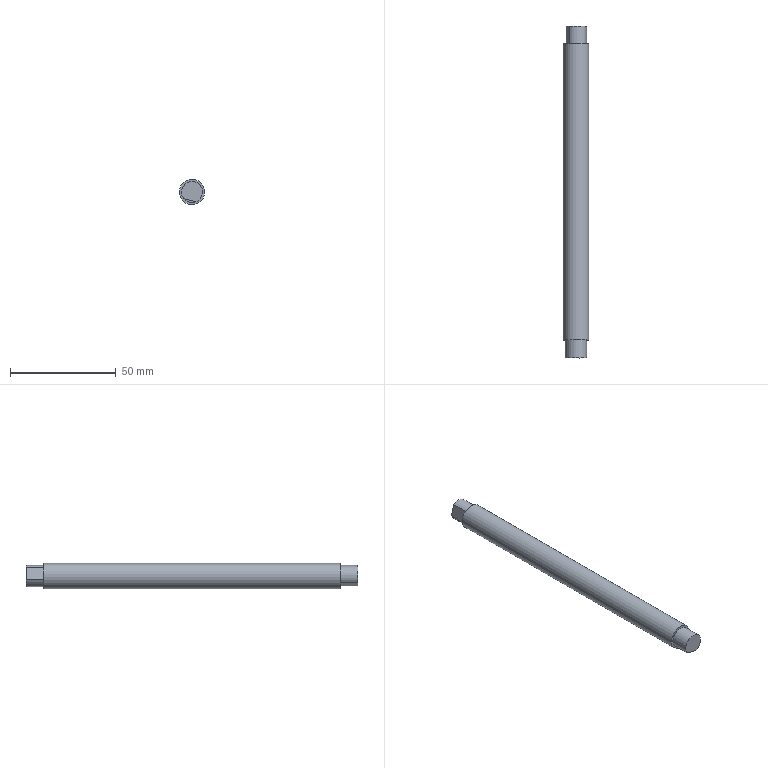Component | NX | LARGE_PULLEY_SHAFT | 1 solid | 13 faces | box 12 x 157 x 12 mm | volume 17079 mm3 | plane 8 | cylinder 5 | commonest cylinder face diameters 10 x4 12 x1
STEP:
#1=CARTESIAN_POINT('',(0.,0.,0.));
#2=DIRECTION('',(0.,0.,1.));
#3=DIRECTION('',(1.,0.,0.));
#4=AXIS2_PLACEMENT_3D('',#1,#2,#3);
#5=CARTESIAN_POINT('',(151.363,-70.,106.36));
#6=VERTEX_POINT('',#5);
#7=CARTESIAN_POINT('',(145.567,-70.,107.913));
#8=VERTEX_POINT('',#7);
#9=CARTESIAN_POINT('',(149.5,-70.,111.));
#10=DIRECTION('',(0.,-1.,0.));
#11=DIRECTION('',(0.2588,0.,0.9659));
#12=AXIS2_PLACEMENT_3D('',#9,#10,#11);
#13=CIRCLE('',#12,5.);
#14=CARTESIAN_POINT('',(149.5,-70.,111.));
#15=DIRECTION('',(0.,-1.,0.));
#16=DIRECTION('',(0.2588,0.,0.9659));
#17=AXIS2_PLACEMENT_3D('',#14,#15,#16);
#18=CYLINDRICAL_SURFACE('',#17,5.);
#19=CARTESIAN_POINT('',(-0.,0.));
#20=DIRECTION('',(1.,0.));
#21=VECTOR('',#20,1.);
#22=LINE('',#19,#21);
#23=(GEOMETRIC_REPRESENTATION_CONTEXT(2)PARAMETRIC_REPRESENTATION_CONTEXT()REPRESENTATION_CONTEXT('',''));
#24=DEFINITIONAL_REPRESENTATION('',(#22),#23);
#25=PCURVE('',#18,#24);
#26=CARTESIAN_POINT('',(149.5,-70.,111.));
#27=DIRECTION('',(0.,-1.,0.));
#28=DIRECTION('',(0.2588,0.,0.9659));
#29=AXIS2_PLACEMENT_3D('',#26,#27,#28);
#30=PLANE('',#29);
#31=CARTESIAN_POINT('',(0.,0.));
#32=DIRECTION('',(1.,0.));
#33=AXIS2_PLACEMENT_2D('',#31,#32);
#34=CIRCLE('',#33,5.);
#35=(GEOMETRIC_REPRESENTATION_CONTEXT(2)PARAMETRIC_REPRESENTATION_CONTEXT()REPRESENTATION_CONTEXT('',''));
#36=DEFINITIONAL_REPRESENTATION('',(#34),#35);
#37=PCURVE('',#30,#36);
#38=SURFACE_CURVE('',#13,(#25,#37),.PCURVE_S1.);
#39=EDGE_CURVE('',#6,#8,#38,.T.);
#40=ORIENTED_EDGE('',*,*,#39,.T.);
#41=CARTESIAN_POINT('',(145.567,-78.5,107.913));
#42=VERTEX_POINT('',#41);
#43=CARTESIAN_POINT('',(145.567,-67.5,107.913));
#44=DIRECTION('',(0.,-1.,0.));
#45=VECTOR('',#44,1.);
#46=LINE('',#43,#45);
#47=CARTESIAN_POINT('',(8.781,-2.5));
#48=DIRECTION('',(0.,1.));
#49=VECTOR('',#48,1.);
#50=LINE('',#47,#49);
#51=(GEOMETRIC_REPRESENTATION_CONTEXT(2)PARAMETRIC_REPRESENTATION_CONTEXT()REPRESENTATION_CONTEXT('',''));
#52=DEFINITIONAL_REPRESENTATION('',(#50),#51);
#53=PCURVE('',#18,#52);
#54=CARTESIAN_POINT('',(145.567,-67.5,107.913));
#55=DIRECTION('',(-0.2588,0.,-0.9659));
#56=DIRECTION('',(-0.9659,0.,0.2588));
#57=AXIS2_PLACEMENT_3D('',#54,#55,#56);
#58=PLANE('',#57);
#59=CARTESIAN_POINT('',(0.,0.));
#60=DIRECTION('',(0.,-1.));
#61=VECTOR('',#60,1.);
#62=LINE('',#59,#61);
#63=(GEOMETRIC_REPRESENTATION_CONTEXT(2)PARAMETRIC_REPRESENTATION_CONTEXT()REPRESENTATION_CONTEXT('',''));
#64=DEFINITIONAL_REPRESENTATION('',(#62),#63);
#65=PCURVE('',#58,#64);
#66=SURFACE_CURVE('',#46,(#53,#65),.PCURVE_S1.);
#67=EDGE_CURVE('',#8,#42,#66,.T.);
#68=ORIENTED_EDGE('',*,*,#67,.T.);
#69=CARTESIAN_POINT('',(151.363,-78.5,106.36));
#70=VERTEX_POINT('',#69);
#71=CARTESIAN_POINT('',(149.5,-78.5,111.));
#72=DIRECTION('',(0.,-1.,0.));
#73=DIRECTION('',(0.2588,0.,0.9659));
#74=AXIS2_PLACEMENT_3D('',#71,#72,#73);
#75=CIRCLE('',#74,5.);
#76=CARTESIAN_POINT('',(-0.,8.5));
#77=DIRECTION('',(1.,0.));
#78=VECTOR('',#77,1.);
#79=LINE('',#76,#78);
#80=(GEOMETRIC_REPRESENTATION_CONTEXT(2)PARAMETRIC_REPRESENTATION_CONTEXT()REPRESENTATION_CONTEXT('',''));
#81=DEFINITIONAL_REPRESENTATION('',(#79),#80);
#82=PCURVE('',#18,#81);
#83=CARTESIAN_POINT('',(149.5,-78.5,111.));
#84=DIRECTION('',(0.,-1.,0.));
#85=DIRECTION('',(0.2588,0.,0.9659));
#86=AXIS2_PLACEMENT_3D('',#83,#84,#85);
#87=PLANE('',#86);
#88=CARTESIAN_POINT('',(0.,0.));
#89=DIRECTION('',(1.,0.));
#90=AXIS2_PLACEMENT_2D('',#88,#89);
#91=CIRCLE('',#90,5.);
#92=(GEOMETRIC_REPRESENTATION_CONTEXT(2)PARAMETRIC_REPRESENTATION_CONTEXT()REPRESENTATION_CONTEXT('',''));
#93=DEFINITIONAL_REPRESENTATION('',(#91),#92);
#94=PCURVE('',#87,#93);
#95=SURFACE_CURVE('',#75,(#82,#94),.PCURVE_S1.);
#96=EDGE_CURVE('',#70,#42,#95,.T.);
#97=ORIENTED_EDGE('',*,*,#96,.F.);
#98=CARTESIAN_POINT('',(151.363,-67.5,106.36));
#99=DIRECTION('',(0.,1.,0.));
#100=VECTOR('',#99,1.);
#101=LINE('',#98,#100);
#102=CARTESIAN_POINT('',(3.785,-2.5));
#103=DIRECTION('',(0.,-1.));
#104=VECTOR('',#103,1.);
#105=LINE('',#102,#104);
#106=(GEOMETRIC_REPRESENTATION_CONTEXT(2)PARAMETRIC_REPRESENTATION_CONTEXT()REPRESENTATION_CONTEXT('',''));
#107=DEFINITIONAL_REPRESENTATION('',(#105),#106);
#108=PCURVE('',#18,#107);
#109=CARTESIAN_POINT('',(-6.,0.));
#110=DIRECTION('',(0.,1.));
#111=VECTOR('',#110,1.);
#112=LINE('',#109,#111);
#113=(GEOMETRIC_REPRESENTATION_CONTEXT(2)PARAMETRIC_REPRESENTATION_CONTEXT()REPRESENTATION_CONTEXT('',''));
#114=DEFINITIONAL_REPRESENTATION('',(#112),#113);
#115=PCURVE('',#58,#114);
#116=SURFACE_CURVE('',#101,(#108,#115),.PCURVE_S1.);
#117=EDGE_CURVE('',#70,#6,#116,.T.);
#118=ORIENTED_EDGE('',*,*,#117,.T.);
#119=EDGE_LOOP('',(#40,#68,#97,#118));
#120=FACE_BOUND('',#119,.T.);
#121=ADVANCED_FACE('',(#120),#18,.T.);
#122=CARTESIAN_POINT('',(144.86,70.,109.137));
#123=VERTEX_POINT('',#122);
#124=CARTESIAN_POINT('',(146.413,70.,114.933));
#125=VERTEX_POINT('',#124);
#126=CARTESIAN_POINT('',(149.5,70.,111.));
#127=DIRECTION('',(0.,1.,0.));
#128=DIRECTION('',(-0.2588,0.,-0.9659));
#129=AXIS2_PLACEMENT_3D('',#126,#127,#128);
#130=CIRCLE('',#129,5.);
#131=CARTESIAN_POINT('',(149.5,70.,111.));
#132=DIRECTION('',(0.,1.,0.));
#133=DIRECTION('',(-0.2588,0.,-0.9659));
#134=AXIS2_PLACEMENT_3D('',#131,#132,#133);
#135=PLANE('',#134);
#136=CARTESIAN_POINT('',(0.,0.));
#137=DIRECTION('',(1.,-0.));
#138=AXIS2_PLACEMENT_2D('',#136,#137);
#139=CIRCLE('',#138,5.);
#140=(GEOMETRIC_REPRESENTATION_CONTEXT(2)PARAMETRIC_REPRESENTATION_CONTEXT()REPRESENTATION_CONTEXT('',''));
#141=DEFINITIONAL_REPRESENTATION('',(#139),#140);
#142=PCURVE('',#135,#141);
#143=CARTESIAN_POINT('',(149.5,67.5,111.));
#144=DIRECTION('',(0.,1.,0.));
#145=DIRECTION('',(-0.2588,0.,-0.9659));
#146=AXIS2_PLACEMENT_3D('',#143,#144,#145);
#147=CYLINDRICAL_SURFACE('',#146,5.);
#148=CARTESIAN_POINT('',(0.,2.5));
#149=DIRECTION('',(1.,0.));
#150=VECTOR('',#149,1.);
#151=LINE('',#148,#150);
#152=(GEOMETRIC_REPRESENTATION_CONTEXT(2)PARAMETRIC_REPRESENTATION_CONTEXT()REPRESENTATION_CONTEXT('',''));
#153=DEFINITIONAL_REPRESENTATION('',(#151),#152);
#154=PCURVE('',#147,#153);
#155=SURFACE_CURVE('',#130,(#142,#154),.PCURVE_S1.);
#156=EDGE_CURVE('',#123,#125,#155,.T.);
#157=ORIENTED_EDGE('',*,*,#156,.F.);
#158=CARTESIAN_POINT('',(149.5,70.,111.));
#159=DIRECTION('',(0.,1.,0.));
#160=DIRECTION('',(-0.2588,0.,-0.9659));
#161=AXIS2_PLACEMENT_3D('',#158,#159,#160);
#162=CIRCLE('',#161,5.);
#163=CARTESIAN_POINT('',(0.,0.));
#164=DIRECTION('',(1.,-0.));
#165=AXIS2_PLACEMENT_2D('',#163,#164);
#166=CIRCLE('',#165,5.);
#167=(GEOMETRIC_REPRESENTATION_CONTEXT(2)PARAMETRIC_REPRESENTATION_CONTEXT()REPRESENTATION_CONTEXT('',''));
#168=DEFINITIONAL_REPRESENTATION('',(#166),#167);
#169=PCURVE('',#135,#168);
#170=CARTESIAN_POINT('',(149.5,70.,111.));
#171=DIRECTION('',(0.,1.,0.));
#172=DIRECTION('',(-0.2588,0.,-0.9659));
#173=AXIS2_PLACEMENT_3D('',#170,#171,#172);
#174=CYLINDRICAL_SURFACE('',#173,5.);
#175=CARTESIAN_POINT('',(-0.,0.));
#176=DIRECTION('',(1.,0.));
#177=VECTOR('',#176,1.);
#178=LINE('',#175,#177);
#179=(GEOMETRIC_REPRESENTATION_CONTEXT(2)PARAMETRIC_REPRESENTATION_CONTEXT()REPRESENTATION_CONTEXT('',''));
#180=DEFINITIONAL_REPRESENTATION('',(#178),#179);
#181=PCURVE('',#174,#180);
#182=SURFACE_CURVE('',#162,(#169,#181),.PCURVE_S1.);
#183=EDGE_CURVE('',#125,#123,#182,.T.);
#184=ORIENTED_EDGE('',*,*,#183,.F.);
#185=EDGE_LOOP('',(#157,#184));
#186=FACE_BOUND('',#185,.T.);
#187=CARTESIAN_POINT('',(147.947,70.,105.204));
#188=VERTEX_POINT('',#187);
#189=CARTESIAN_POINT('',(149.5,70.,111.));
#190=DIRECTION('',(0.,-1.,0.));
#191=DIRECTION('',(-0.2588,0.,-0.9659));
#192=AXIS2_PLACEMENT_3D('',#189,#190,#191);
#193=CIRCLE('',#192,6.);
#194=CARTESIAN_POINT('',(6.,0.));
#195=CARTESIAN_POINT('',(6.,-10.392));
#196=CARTESIAN_POINT('',(-3.,-5.196));
#197=CARTESIAN_POINT('',(-12.,-0.));
#198=CARTESIAN_POINT('',(-3.,5.196));
#199=CARTESIAN_POINT('',(6.,10.392));
#200=CARTESIAN_POINT('',(6.,0.));
#201=(BOUNDED_CURVE()B_SPLINE_CURVE(2,(#194,#195,#196,#197,#198,#199,#200),.UNSPECIFIED.,.T.,.F.)B_SPLINE_CURVE_WITH_KNOTS((1,2,2,2,2,1),(-2.094,0.,2.094,4.189,6.283,8.378),.UNSPECIFIED.)CURVE()GEOMETRIC_REPRESENTATION_ITEM()RATIONAL_B_SPLINE_CURVE((1.,0.5,1.,0.5,1.,0.5,1.))REPRESENTATION_ITEM(''));
#202=(GEOMETRIC_REPRESENTATION_CONTEXT(2)PARAMETRIC_REPRESENTATION_CONTEXT()REPRESENTATION_CONTEXT('',''));
#203=DEFINITIONAL_REPRESENTATION('',(#201),#202);
#204=PCURVE('',#135,#203);
#205=CARTESIAN_POINT('',(149.5,-70.,111.));
#206=DIRECTION('',(0.,1.,0.));
#207=DIRECTION('',(-0.2588,0.,-0.9659));
#208=AXIS2_PLACEMENT_3D('',#205,#206,#207);
#209=CYLINDRICAL_SURFACE('',#208,6.);
#210=CARTESIAN_POINT('',(6.283,140.));
#211=DIRECTION('',(-1.,0.));
#212=VECTOR('',#211,1.);
#213=LINE('',#210,#212);
#214=(GEOMETRIC_REPRESENTATION_CONTEXT(2)PARAMETRIC_REPRESENTATION_CONTEXT()REPRESENTATION_CONTEXT('',''));
#215=DEFINITIONAL_REPRESENTATION('',(#213),#214);
#216=PCURVE('',#209,#215);
#217=SURFACE_CURVE('',#193,(#204,#216),.PCURVE_S1.);
#218=EDGE_CURVE('',#188,#188,#217,.T.);
#219=ORIENTED_EDGE('',*,*,#218,.F.);
#220=EDGE_LOOP('',(#219));
#221=FACE_BOUND('',#220,.T.);
#222=ADVANCED_FACE('',(#186,#221),#135,.T.);
#223=CARTESIAN_POINT('',(149.5,-70.,111.));
#224=DIRECTION('',(0.,-1.,0.));
#225=DIRECTION('',(0.2588,0.,0.9659));
#226=AXIS2_PLACEMENT_3D('',#223,#224,#225);
#227=CIRCLE('',#226,5.);
#228=CARTESIAN_POINT('',(0.,0.));
#229=DIRECTION('',(1.,0.));
#230=AXIS2_PLACEMENT_2D('',#228,#229);
#231=CIRCLE('',#230,5.);
#232=(GEOMETRIC_REPRESENTATION_CONTEXT(2)PARAMETRIC_REPRESENTATION_CONTEXT()REPRESENTATION_CONTEXT('',''));
#233=DEFINITIONAL_REPRESENTATION('',(#231),#232);
#234=PCURVE('',#30,#233);
#235=CARTESIAN_POINT('',(149.5,-67.5,111.));
#236=DIRECTION('',(0.,-1.,0.));
#237=DIRECTION('',(0.2588,0.,0.9659));
#238=AXIS2_PLACEMENT_3D('',#235,#236,#237);
#239=CYLINDRICAL_SURFACE('',#238,5.);
#240=CARTESIAN_POINT('',(-0.,2.5));
#241=DIRECTION('',(1.,0.));
#242=VECTOR('',#241,1.);
#243=LINE('',#240,#242);
#244=(GEOMETRIC_REPRESENTATION_CONTEXT(2)PARAMETRIC_REPRESENTATION_CONTEXT()REPRESENTATION_CONTEXT('',''));
#245=DEFINITIONAL_REPRESENTATION('',(#243),#244);
#246=PCURVE('',#239,#245);
#247=SURFACE_CURVE('',#227,(#234,#246),.PCURVE_S1.);
#248=EDGE_CURVE('',#8,#6,#247,.T.);
#249=ORIENTED_EDGE('',*,*,#248,.F.);
#250=ORIENTED_EDGE('',*,*,#39,.F.);
#251=EDGE_LOOP('',(#249,#250));
#252=FACE_BOUND('',#251,.T.);
#253=CARTESIAN_POINT('',(147.947,-70.,105.204));
#254=VERTEX_POINT('',#253);
#255=CARTESIAN_POINT('',(149.5,-70.,111.));
#256=DIRECTION('',(0.,1.,0.));
#257=DIRECTION('',(-0.2588,0.,-0.9659));
#258=AXIS2_PLACEMENT_3D('',#255,#256,#257);
#259=CIRCLE('',#258,6.);
#260=CARTESIAN_POINT('',(-6.,0.));
#261=CARTESIAN_POINT('',(-6.,10.392));
#262=CARTESIAN_POINT('',(3.,5.196));
#263=CARTESIAN_POINT('',(12.,-0.));
#264=CARTESIAN_POINT('',(3.,-5.196));
#265=CARTESIAN_POINT('',(-6.,-10.392));
#266=CARTESIAN_POINT('',(-6.,0.));
#267=(BOUNDED_CURVE()B_SPLINE_CURVE(2,(#260,#261,#262,#263,#264,#265,#266),.UNSPECIFIED.,.T.,.F.)B_SPLINE_CURVE_WITH_KNOTS((1,2,2,2,2,1),(-2.094,0.,2.094,4.189,6.283,8.378),.UNSPECIFIED.)CURVE()GEOMETRIC_REPRESENTATION_ITEM()RATIONAL_B_SPLINE_CURVE((1.,0.5,1.,0.5,1.,0.5,1.))REPRESENTATION_ITEM(''));
#268=(GEOMETRIC_REPRESENTATION_CONTEXT(2)PARAMETRIC_REPRESENTATION_CONTEXT()REPRESENTATION_CONTEXT('',''));
#269=DEFINITIONAL_REPRESENTATION('',(#267),#268);
#270=PCURVE('',#30,#269);
#271=CARTESIAN_POINT('',(0.,0.));
#272=DIRECTION('',(1.,0.));
#273=VECTOR('',#272,1.);
#274=LINE('',#271,#273);
#275=(GEOMETRIC_REPRESENTATION_CONTEXT(2)PARAMETRIC_REPRESENTATION_CONTEXT()REPRESENTATION_CONTEXT('',''));
#276=DEFINITIONAL_REPRESENTATION('',(#274),#275);
#277=PCURVE('',#209,#276);
#278=SURFACE_CURVE('',#259,(#270,#277),.PCURVE_S1.);
#279=EDGE_CURVE('',#254,#254,#278,.T.);
#280=ORIENTED_EDGE('',*,*,#279,.F.);
#281=EDGE_LOOP('',(#280));
#282=FACE_BOUND('',#281,.T.);
#283=ADVANCED_FACE('',(#252,#282),#30,.T.);
#284=ORIENTED_EDGE('',*,*,#218,.T.);
#285=CARTESIAN_POINT('',(147.947,-70.,105.204));
#286=CARTESIAN_POINT('',(147.947,70.,105.204));
#287=B_SPLINE_CURVE_WITH_KNOTS('',1,(#285,#286),.UNSPECIFIED.,.F.,.F.,(2,2),(0.,140.),.PIECEWISE_BEZIER_KNOTS.);
#288=CARTESIAN_POINT('',(0.,0.));
#289=DIRECTION('',(0.,1.));
#290=VECTOR('',#289,1.);
#291=LINE('',#288,#290);
#292=(GEOMETRIC_REPRESENTATION_CONTEXT(2)PARAMETRIC_REPRESENTATION_CONTEXT()REPRESENTATION_CONTEXT('',''));
#293=DEFINITIONAL_REPRESENTATION('',(#291),#292);
#294=PCURVE('',#209,#293);
#295=CARTESIAN_POINT('',(6.283,0.));
#296=DIRECTION('',(0.,1.));
#297=VECTOR('',#296,1.);
#298=LINE('',#295,#297);
#299=(GEOMETRIC_REPRESENTATION_CONTEXT(2)PARAMETRIC_REPRESENTATION_CONTEXT()REPRESENTATION_CONTEXT('',''));
#300=DEFINITIONAL_REPRESENTATION('',(#298),#299);
#301=PCURVE('',#209,#300);
#302=SEAM_CURVE('',#287,(#294,#301),.PCURVE_S1.);
#303=EDGE_CURVE('',#254,#188,#302,.T.);
#304=ORIENTED_EDGE('',*,*,#303,.F.);
#305=ORIENTED_EDGE('',*,*,#279,.T.);
#306=ORIENTED_EDGE('',*,*,#303,.T.);
#307=EDGE_LOOP('',(#284,#304,#305,#306));
#308=FACE_BOUND('',#307,.T.);
#309=ADVANCED_FACE('',(#308),#209,.T.);
#310=CARTESIAN_POINT('',(146.413,78.5,114.933));
#311=VERTEX_POINT('',#310);
#312=CARTESIAN_POINT('',(144.86,78.5,109.137));
#313=VERTEX_POINT('',#312);
#314=CARTESIAN_POINT('',(149.5,78.5,111.));
#315=DIRECTION('',(0.,1.,0.));
#316=DIRECTION('',(-0.2588,0.,-0.9659));
#317=AXIS2_PLACEMENT_3D('',#314,#315,#316);
#318=CIRCLE('',#317,5.);
#319=CARTESIAN_POINT('',(149.5,78.5,111.));
#320=DIRECTION('',(0.,1.,0.));
#321=DIRECTION('',(-0.2588,0.,-0.9659));
#322=AXIS2_PLACEMENT_3D('',#319,#320,#321);
#323=PLANE('',#322);
#324=CARTESIAN_POINT('',(0.,0.));
#325=DIRECTION('',(1.,-0.));
#326=AXIS2_PLACEMENT_2D('',#324,#325);
#327=CIRCLE('',#326,5.);
#328=(GEOMETRIC_REPRESENTATION_CONTEXT(2)PARAMETRIC_REPRESENTATION_CONTEXT()REPRESENTATION_CONTEXT('',''));
#329=DEFINITIONAL_REPRESENTATION('',(#327),#328);
#330=PCURVE('',#323,#329);
#331=CARTESIAN_POINT('',(-0.,8.5));
#332=DIRECTION('',(1.,0.));
#333=VECTOR('',#332,1.);
#334=LINE('',#331,#333);
#335=(GEOMETRIC_REPRESENTATION_CONTEXT(2)PARAMETRIC_REPRESENTATION_CONTEXT()REPRESENTATION_CONTEXT('',''));
#336=DEFINITIONAL_REPRESENTATION('',(#334),#335);
#337=PCURVE('',#174,#336);
#338=SURFACE_CURVE('',#318,(#330,#337),.PCURVE_S1.);
#339=EDGE_CURVE('',#311,#313,#338,.T.);
#340=ORIENTED_EDGE('',*,*,#339,.T.);
#341=CARTESIAN_POINT('',(144.86,78.5,109.137));
#342=DIRECTION('',(0.2588,0.,0.9659));
#343=VECTOR('',#342,1.);
#344=LINE('',#341,#343);
#345=CARTESIAN_POINT('',(3.,4.));
#346=DIRECTION('',(-1.,0.));
#347=VECTOR('',#346,1.);
#348=LINE('',#345,#347);
#349=(GEOMETRIC_REPRESENTATION_CONTEXT(2)PARAMETRIC_REPRESENTATION_CONTEXT()REPRESENTATION_CONTEXT('',''));
#350=DEFINITIONAL_REPRESENTATION('',(#348),#349);
#351=PCURVE('',#323,#350);
#352=CARTESIAN_POINT('',(144.86,67.5,109.137));
#353=DIRECTION('',(-0.9659,0.,0.2588));
#354=DIRECTION('',(0.2588,0.,0.9659));
#355=AXIS2_PLACEMENT_3D('',#352,#353,#354);
#356=PLANE('',#355);
#357=CARTESIAN_POINT('',(0.,11.));
#358=DIRECTION('',(1.,0.));
#359=VECTOR('',#358,1.);
#360=LINE('',#357,#359);
#361=(GEOMETRIC_REPRESENTATION_CONTEXT(2)PARAMETRIC_REPRESENTATION_CONTEXT()REPRESENTATION_CONTEXT('',''));
#362=DEFINITIONAL_REPRESENTATION('',(#360),#361);
#363=PCURVE('',#356,#362);
#364=SURFACE_CURVE('',#344,(#351,#363),.PCURVE_S1.);
#365=EDGE_CURVE('',#313,#311,#364,.T.);
#366=ORIENTED_EDGE('',*,*,#365,.T.);
#367=EDGE_LOOP('',(#340,#366));
#368=FACE_BOUND('',#367,.T.);
#369=ADVANCED_FACE('',(#368),#323,.T.);
#370=CARTESIAN_POINT('',(144.86,67.5,109.137));
#371=DIRECTION('',(0.,-1.,0.));
#372=VECTOR('',#371,1.);
#373=LINE('',#370,#372);
#374=CARTESIAN_POINT('',(7.21,-2.5));
#375=DIRECTION('',(0.,-1.));
#376=VECTOR('',#375,1.);
#377=LINE('',#374,#376);
#378=(GEOMETRIC_REPRESENTATION_CONTEXT(2)PARAMETRIC_REPRESENTATION_CONTEXT()REPRESENTATION_CONTEXT('',''));
#379=DEFINITIONAL_REPRESENTATION('',(#377),#378);
#380=PCURVE('',#174,#379);
#381=CARTESIAN_POINT('',(0.,0.));
#382=DIRECTION('',(0.,-1.));
#383=VECTOR('',#382,1.);
#384=LINE('',#381,#383);
#385=(GEOMETRIC_REPRESENTATION_CONTEXT(2)PARAMETRIC_REPRESENTATION_CONTEXT()REPRESENTATION_CONTEXT('',''));
#386=DEFINITIONAL_REPRESENTATION('',(#384),#385);
#387=PCURVE('',#356,#386);
#388=SURFACE_CURVE('',#373,(#380,#387),.PCURVE_S1.);
#389=EDGE_CURVE('',#313,#123,#388,.T.);
#390=ORIENTED_EDGE('',*,*,#389,.F.);
#391=ORIENTED_EDGE('',*,*,#339,.F.);
#392=CARTESIAN_POINT('',(146.413,67.5,114.933));
#393=DIRECTION('',(0.,1.,0.));
#394=VECTOR('',#393,1.);
#395=LINE('',#392,#394);
#396=CARTESIAN_POINT('',(2.214,-2.5));
#397=DIRECTION('',(0.,1.));
#398=VECTOR('',#397,1.);
#399=LINE('',#396,#398);
#400=(GEOMETRIC_REPRESENTATION_CONTEXT(2)PARAMETRIC_REPRESENTATION_CONTEXT()REPRESENTATION_CONTEXT('',''));
#401=DEFINITIONAL_REPRESENTATION('',(#399),#400);
#402=PCURVE('',#174,#401);
#403=CARTESIAN_POINT('',(6.,0.));
#404=DIRECTION('',(0.,1.));
#405=VECTOR('',#404,1.);
#406=LINE('',#403,#405);
#407=(GEOMETRIC_REPRESENTATION_CONTEXT(2)PARAMETRIC_REPRESENTATION_CONTEXT()REPRESENTATION_CONTEXT('',''));
#408=DEFINITIONAL_REPRESENTATION('',(#406),#407);
#409=PCURVE('',#356,#408);
#410=SURFACE_CURVE('',#395,(#402,#409),.PCURVE_S1.);
#411=EDGE_CURVE('',#125,#311,#410,.T.);
#412=ORIENTED_EDGE('',*,*,#411,.F.);
#413=ORIENTED_EDGE('',*,*,#183,.T.);
#414=EDGE_LOOP('',(#390,#391,#412,#413));
#415=FACE_BOUND('',#414,.T.);
#416=ADVANCED_FACE('',(#415),#174,.T.);
#417=ORIENTED_EDGE('',*,*,#96,.T.);
#418=CARTESIAN_POINT('',(145.567,-78.5,107.913));
#419=DIRECTION('',(0.9659,0.,-0.2588));
#420=VECTOR('',#419,1.);
#421=LINE('',#418,#420);
#422=CARTESIAN_POINT('',(-4.,3.));
#423=DIRECTION('',(-0.,-1.));
#424=VECTOR('',#423,1.);
#425=LINE('',#422,#424);
#426=(GEOMETRIC_REPRESENTATION_CONTEXT(2)PARAMETRIC_REPRESENTATION_CONTEXT()REPRESENTATION_CONTEXT('',''));
#427=DEFINITIONAL_REPRESENTATION('',(#425),#426);
#428=PCURVE('',#87,#427);
#429=CARTESIAN_POINT('',(0.,-11.));
#430=DIRECTION('',(-1.,0.));
#431=VECTOR('',#430,1.);
#432=LINE('',#429,#431);
#433=(GEOMETRIC_REPRESENTATION_CONTEXT(2)PARAMETRIC_REPRESENTATION_CONTEXT()REPRESENTATION_CONTEXT('',''));
#434=DEFINITIONAL_REPRESENTATION('',(#432),#433);
#435=PCURVE('',#58,#434);
#436=SURFACE_CURVE('',#421,(#428,#435),.PCURVE_S1.);
#437=EDGE_CURVE('',#42,#70,#436,.T.);
#438=ORIENTED_EDGE('',*,*,#437,.T.);
#439=EDGE_LOOP('',(#417,#438));
#440=FACE_BOUND('',#439,.T.);
#441=ADVANCED_FACE('',(#440),#87,.T.);
#442=CARTESIAN_POINT('',(144.86,67.5,109.137));
#443=VERTEX_POINT('',#442);
#444=CARTESIAN_POINT('',(144.86,67.5,109.137));
#445=DIRECTION('',(0.,1.,0.));
#446=VECTOR('',#445,1.);
#447=LINE('',#444,#446);
#448=CARTESIAN_POINT('',(0.9273,0.));
#449=DIRECTION('',(0.,1.));
#450=VECTOR('',#449,1.);
#451=LINE('',#448,#450);
#452=(GEOMETRIC_REPRESENTATION_CONTEXT(2)PARAMETRIC_REPRESENTATION_CONTEXT()REPRESENTATION_CONTEXT('',''));
#453=DEFINITIONAL_REPRESENTATION('',(#451),#452);
#454=PCURVE('',#147,#453);
#455=CARTESIAN_POINT('',(0.,0.));
#456=DIRECTION('',(0.,1.));
#457=VECTOR('',#456,1.);
#458=LINE('',#455,#457);
#459=(GEOMETRIC_REPRESENTATION_CONTEXT(2)PARAMETRIC_REPRESENTATION_CONTEXT()REPRESENTATION_CONTEXT('',''));
#460=DEFINITIONAL_REPRESENTATION('',(#458),#459);
#461=PCURVE('',#356,#460);
#462=SURFACE_CURVE('',#447,(#454,#461),.PCURVE_S1.);
#463=EDGE_CURVE('',#443,#123,#462,.T.);
#464=ORIENTED_EDGE('',*,*,#463,.F.);
#465=CARTESIAN_POINT('',(146.413,67.5,114.933));
#466=VERTEX_POINT('',#465);
#467=CARTESIAN_POINT('',(149.5,67.5,111.));
#468=DIRECTION('',(0.,1.,0.));
#469=DIRECTION('',(-0.2588,0.,-0.9659));
#470=AXIS2_PLACEMENT_3D('',#467,#468,#469);
#471=CIRCLE('',#470,5.);
#472=CARTESIAN_POINT('',(0.,0.));
#473=DIRECTION('',(1.,0.));
#474=VECTOR('',#473,1.);
#475=LINE('',#472,#474);
#476=(GEOMETRIC_REPRESENTATION_CONTEXT(2)PARAMETRIC_REPRESENTATION_CONTEXT()REPRESENTATION_CONTEXT('',''));
#477=DEFINITIONAL_REPRESENTATION('',(#475),#476);
#478=PCURVE('',#147,#477);
#479=CARTESIAN_POINT('',(149.5,67.5,111.));
#480=DIRECTION('',(0.,-1.,0.));
#481=DIRECTION('',(0.2588,0.,0.9659));
#482=AXIS2_PLACEMENT_3D('',#479,#480,#481);
#483=PLANE('',#482);
#484=CARTESIAN_POINT('',(-5.,-0.));
#485=CARTESIAN_POINT('',(-5.,8.66));
#486=CARTESIAN_POINT('',(2.5,4.33));
#487=CARTESIAN_POINT('',(10.,0.));
#488=CARTESIAN_POINT('',(2.5,-4.33));
#489=CARTESIAN_POINT('',(-5.,-8.66));
#490=CARTESIAN_POINT('',(-5.,-0.));
#491=(BOUNDED_CURVE()B_SPLINE_CURVE(2,(#484,#485,#486,#487,#488,#489,#490),.UNSPECIFIED.,.T.,.F.)B_SPLINE_CURVE_WITH_KNOTS((1,2,2,2,2,1),(-2.094,0.,2.094,4.189,6.283,8.378),.UNSPECIFIED.)CURVE()GEOMETRIC_REPRESENTATION_ITEM()RATIONAL_B_SPLINE_CURVE((1.,0.5,1.,0.5,1.,0.5,1.))REPRESENTATION_ITEM(''));
#492=(GEOMETRIC_REPRESENTATION_CONTEXT(2)PARAMETRIC_REPRESENTATION_CONTEXT()REPRESENTATION_CONTEXT('',''));
#493=DEFINITIONAL_REPRESENTATION('',(#491),#492);
#494=PCURVE('',#483,#493);
#495=SURFACE_CURVE('',#471,(#478,#494),.PCURVE_S1.);
#496=EDGE_CURVE('',#443,#466,#495,.T.);
#497=ORIENTED_EDGE('',*,*,#496,.T.);
#498=CARTESIAN_POINT('',(146.413,67.5,114.933));
#499=DIRECTION('',(0.,-1.,0.));
#500=VECTOR('',#499,1.);
#501=LINE('',#498,#500);
#502=CARTESIAN_POINT('',(2.214,0.));
#503=DIRECTION('',(0.,-1.));
#504=VECTOR('',#503,1.);
#505=LINE('',#502,#504);
#506=(GEOMETRIC_REPRESENTATION_CONTEXT(2)PARAMETRIC_REPRESENTATION_CONTEXT()REPRESENTATION_CONTEXT('',''));
#507=DEFINITIONAL_REPRESENTATION('',(#505),#506);
#508=PCURVE('',#147,#507);
#509=CARTESIAN_POINT('',(6.,0.));
#510=DIRECTION('',(0.,-1.));
#511=VECTOR('',#510,1.);
#512=LINE('',#509,#511);
#513=(GEOMETRIC_REPRESENTATION_CONTEXT(2)PARAMETRIC_REPRESENTATION_CONTEXT()REPRESENTATION_CONTEXT('',''));
#514=DEFINITIONAL_REPRESENTATION('',(#512),#513);
#515=PCURVE('',#356,#514);
#516=SURFACE_CURVE('',#501,(#508,#515),.PCURVE_S1.);
#517=EDGE_CURVE('',#125,#466,#516,.T.);
#518=ORIENTED_EDGE('',*,*,#517,.F.);
#519=ORIENTED_EDGE('',*,*,#156,.F.);
#520=EDGE_LOOP('',(#464,#497,#518,#519));
#521=FACE_BOUND('',#520,.F.);
#522=ADVANCED_FACE('',(#521),#147,.F.);
#523=ORIENTED_EDGE('',*,*,#365,.F.);
#524=ORIENTED_EDGE('',*,*,#389,.T.);
#525=ORIENTED_EDGE('',*,*,#463,.F.);
#526=CARTESIAN_POINT('',(144.86,67.5,109.137));
#527=DIRECTION('',(-0.2588,0.,-0.9659));
#528=VECTOR('',#527,1.);
#529=LINE('',#526,#528);
#530=CARTESIAN_POINT('',(0.,0.));
#531=DIRECTION('',(-1.,0.));
#532=VECTOR('',#531,1.);
#533=LINE('',#530,#532);
#534=(GEOMETRIC_REPRESENTATION_CONTEXT(2)PARAMETRIC_REPRESENTATION_CONTEXT()REPRESENTATION_CONTEXT('',''));
#535=DEFINITIONAL_REPRESENTATION('',(#533),#534);
#536=PCURVE('',#356,#535);
#537=CARTESIAN_POINT('',(-3.,4.));
#538=DIRECTION('',(-1.,0.));
#539=VECTOR('',#538,1.);
#540=LINE('',#537,#539);
#541=(GEOMETRIC_REPRESENTATION_CONTEXT(2)PARAMETRIC_REPRESENTATION_CONTEXT()REPRESENTATION_CONTEXT('',''));
#542=DEFINITIONAL_REPRESENTATION('',(#540),#541);
#543=PCURVE('',#483,#542);
#544=SURFACE_CURVE('',#529,(#536,#543),.PCURVE_S1.);
#545=EDGE_CURVE('',#466,#443,#544,.T.);
#546=ORIENTED_EDGE('',*,*,#545,.F.);
#547=ORIENTED_EDGE('',*,*,#517,.F.);
#548=ORIENTED_EDGE('',*,*,#411,.T.);
#549=EDGE_LOOP('',(#523,#524,#525,#546,#547,#548));
#550=FACE_BOUND('',#549,.T.);
#551=ADVANCED_FACE('',(#550),#356,.T.);
#552=ORIENTED_EDGE('',*,*,#545,.T.);
#553=ORIENTED_EDGE('',*,*,#496,.T.);
#554=EDGE_LOOP('',(#552,#553));
#555=FACE_BOUND('',#554,.T.);
#556=ADVANCED_FACE('',(#555),#483,.F.);
#557=CARTESIAN_POINT('',(145.567,-67.5,107.913));
#558=VERTEX_POINT('',#557);
#559=CARTESIAN_POINT('',(145.567,-67.5,107.913));
#560=DIRECTION('',(0.,1.,0.));
#561=VECTOR('',#560,1.);
#562=LINE('',#559,#561);
#563=CARTESIAN_POINT('',(2.498,0.));
#564=DIRECTION('',(0.,-1.));
#565=VECTOR('',#564,1.);
#566=LINE('',#563,#565);
#567=(GEOMETRIC_REPRESENTATION_CONTEXT(2)PARAMETRIC_REPRESENTATION_CONTEXT()REPRESENTATION_CONTEXT('',''));
#568=DEFINITIONAL_REPRESENTATION('',(#566),#567);
#569=PCURVE('',#239,#568);
#570=CARTESIAN_POINT('',(0.,0.));
#571=DIRECTION('',(0.,1.));
#572=VECTOR('',#571,1.);
#573=LINE('',#570,#572);
#574=(GEOMETRIC_REPRESENTATION_CONTEXT(2)PARAMETRIC_REPRESENTATION_CONTEXT()REPRESENTATION_CONTEXT('',''));
#575=DEFINITIONAL_REPRESENTATION('',(#573),#574);
#576=PCURVE('',#58,#575);
#577=SURFACE_CURVE('',#562,(#569,#576),.PCURVE_S1.);
#578=EDGE_CURVE('',#8,#558,#577,.T.);
#579=ORIENTED_EDGE('',*,*,#578,.T.);
#580=CARTESIAN_POINT('',(151.363,-67.5,106.36));
#581=VERTEX_POINT('',#580);
#582=CARTESIAN_POINT('',(149.5,-67.5,111.));
#583=DIRECTION('',(0.,-1.,0.));
#584=DIRECTION('',(0.2588,0.,0.9659));
#585=AXIS2_PLACEMENT_3D('',#582,#583,#584);
#586=CIRCLE('',#585,5.);
#587=CARTESIAN_POINT('',(-0.,0.));
#588=DIRECTION('',(1.,0.));
#589=VECTOR('',#588,1.);
#590=LINE('',#587,#589);
#591=(GEOMETRIC_REPRESENTATION_CONTEXT(2)PARAMETRIC_REPRESENTATION_CONTEXT()REPRESENTATION_CONTEXT('',''));
#592=DEFINITIONAL_REPRESENTATION('',(#590),#591);
#593=PCURVE('',#239,#592);
#594=CARTESIAN_POINT('',(149.5,-67.5,111.));
#595=DIRECTION('',(0.,1.,0.));
#596=DIRECTION('',(-0.2588,0.,-0.9659));
#597=AXIS2_PLACEMENT_3D('',#594,#595,#596);
#598=PLANE('',#597);
#599=CARTESIAN_POINT('',(-5.,0.));
#600=CARTESIAN_POINT('',(-5.,8.66));
#601=CARTESIAN_POINT('',(2.5,4.33));
#602=CARTESIAN_POINT('',(10.,-0.));
#603=CARTESIAN_POINT('',(2.5,-4.33));
#604=CARTESIAN_POINT('',(-5.,-8.66));
#605=CARTESIAN_POINT('',(-5.,0.));
#606=(BOUNDED_CURVE()B_SPLINE_CURVE(2,(#599,#600,#601,#602,#603,#604,#605),.UNSPECIFIED.,.T.,.F.)B_SPLINE_CURVE_WITH_KNOTS((1,2,2,2,2,1),(-2.094,0.,2.094,4.189,6.283,8.378),.UNSPECIFIED.)CURVE()GEOMETRIC_REPRESENTATION_ITEM()RATIONAL_B_SPLINE_CURVE((1.,0.5,1.,0.5,1.,0.5,1.))REPRESENTATION_ITEM(''));
#607=(GEOMETRIC_REPRESENTATION_CONTEXT(2)PARAMETRIC_REPRESENTATION_CONTEXT()REPRESENTATION_CONTEXT('',''));
#608=DEFINITIONAL_REPRESENTATION('',(#606),#607);
#609=PCURVE('',#598,#608);
#610=SURFACE_CURVE('',#586,(#593,#609),.PCURVE_S1.);
#611=EDGE_CURVE('',#558,#581,#610,.T.);
#612=ORIENTED_EDGE('',*,*,#611,.T.);
#613=CARTESIAN_POINT('',(151.363,-67.5,106.36));
#614=DIRECTION('',(0.,-1.,0.));
#615=VECTOR('',#614,1.);
#616=LINE('',#613,#615);
#617=CARTESIAN_POINT('',(3.785,0.));
#618=DIRECTION('',(0.,1.));
#619=VECTOR('',#618,1.);
#620=LINE('',#617,#619);
#621=(GEOMETRIC_REPRESENTATION_CONTEXT(2)PARAMETRIC_REPRESENTATION_CONTEXT()REPRESENTATION_CONTEXT('',''));
#622=DEFINITIONAL_REPRESENTATION('',(#620),#621);
#623=PCURVE('',#239,#622);
#624=CARTESIAN_POINT('',(-6.,0.));
#625=DIRECTION('',(0.,-1.));
#626=VECTOR('',#625,1.);
#627=LINE('',#624,#626);
#628=(GEOMETRIC_REPRESENTATION_CONTEXT(2)PARAMETRIC_REPRESENTATION_CONTEXT()REPRESENTATION_CONTEXT('',''));
#629=DEFINITIONAL_REPRESENTATION('',(#627),#628);
#630=PCURVE('',#58,#629);
#631=SURFACE_CURVE('',#616,(#623,#630),.PCURVE_S1.);
#632=EDGE_CURVE('',#581,#6,#631,.T.);
#633=ORIENTED_EDGE('',*,*,#632,.T.);
#634=ORIENTED_EDGE('',*,*,#248,.F.);
#635=EDGE_LOOP('',(#579,#612,#633,#634));
#636=FACE_BOUND('',#635,.F.);
#637=ADVANCED_FACE('',(#636),#239,.F.);
#638=ORIENTED_EDGE('',*,*,#437,.F.);
#639=ORIENTED_EDGE('',*,*,#67,.F.);
#640=ORIENTED_EDGE('',*,*,#578,.T.);
#641=CARTESIAN_POINT('',(145.567,-67.5,107.913));
#642=DIRECTION('',(-0.9659,0.,0.2588));
#643=VECTOR('',#642,1.);
#644=LINE('',#641,#643);
#645=CARTESIAN_POINT('',(0.,0.));
#646=DIRECTION('',(1.,0.));
#647=VECTOR('',#646,1.);
#648=LINE('',#645,#647);
#649=(GEOMETRIC_REPRESENTATION_CONTEXT(2)PARAMETRIC_REPRESENTATION_CONTEXT()REPRESENTATION_CONTEXT('',''));
#650=DEFINITIONAL_REPRESENTATION('',(#648),#649);
#651=PCURVE('',#58,#650);
#652=CARTESIAN_POINT('',(4.,3.));
#653=DIRECTION('',(-0.,1.));
#654=VECTOR('',#653,1.);
#655=LINE('',#652,#654);
#656=(GEOMETRIC_REPRESENTATION_CONTEXT(2)PARAMETRIC_REPRESENTATION_CONTEXT()REPRESENTATION_CONTEXT('',''));
#657=DEFINITIONAL_REPRESENTATION('',(#655),#656);
#658=PCURVE('',#598,#657);
#659=SURFACE_CURVE('',#644,(#651,#658),.PCURVE_S1.);
#660=EDGE_CURVE('',#581,#558,#659,.T.);
#661=ORIENTED_EDGE('',*,*,#660,.F.);
#662=ORIENTED_EDGE('',*,*,#632,.T.);
#663=ORIENTED_EDGE('',*,*,#117,.F.);
#664=EDGE_LOOP('',(#638,#639,#640,#661,#662,#663));
#665=FACE_BOUND('',#664,.T.);
#666=ADVANCED_FACE('',(#665),#58,.T.);
#667=ORIENTED_EDGE('',*,*,#611,.T.);
#668=ORIENTED_EDGE('',*,*,#660,.T.);
#669=EDGE_LOOP('',(#667,#668));
#670=FACE_BOUND('',#669,.T.);
#671=ADVANCED_FACE('',(#670),#598,.F.);
#672=CLOSED_SHELL('',(#121,#222,#283,#309,#369,#416,#441,#522,#551,#556,#637,#666,#671));
#673=MANIFOLD_SOLID_BREP('',#672);
#674=(LENGTH_UNIT()NAMED_UNIT(*)SI_UNIT(.MILLI.,.METRE.));
#675=UNCERTAINTY_MEASURE_WITH_UNIT(LENGTH_MEASURE(0.000001),#674,'','');
#676=(NAMED_UNIT(*)PLANE_ANGLE_UNIT()SI_UNIT($,.RADIAN.));
#677=(NAMED_UNIT(*)SI_UNIT($,.STERADIAN.)SOLID_ANGLE_UNIT());
#678=(GEOMETRIC_REPRESENTATION_CONTEXT(3)GLOBAL_UNCERTAINTY_ASSIGNED_CONTEXT((#675))GLOBAL_UNIT_ASSIGNED_CONTEXT((#674,#676,#677))REPRESENTATION_CONTEXT('',''));
#679=ADVANCED_BREP_SHAPE_REPRESENTATION('',(#4,#673),#678);